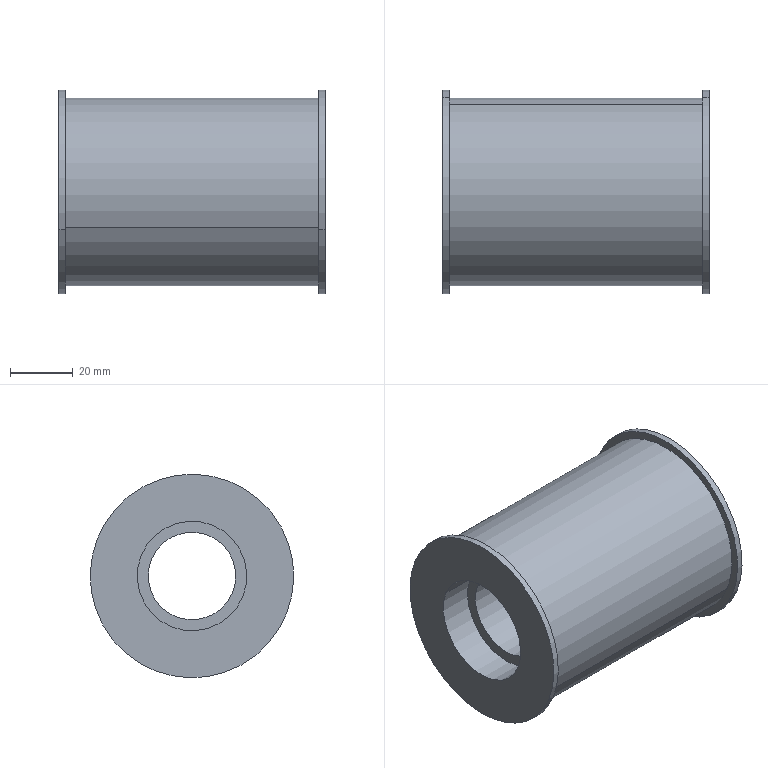Component | SolidWorks | ElectricalBoxAssembly2-1_AuxiliaryWheel-1 | 1 solid | 18 faces | box 85 x 65 x 65 mm | volume 182336 mm3 | cylinder 12 | plane 6 | commonest cylinder face diameters 35 x4 65 x4 28 x2 60 x2
build123d program:
from build123d import *


with BuildPart() as part:
    # Sketch1 → Revolve1 (revolve)
    with BuildSketch(Plane(origin=(0, 0, 0), x_dir=(1, 0, 0), z_dir=(0, 1, 0)), mode=Mode.PRIVATE) as revolve1_sk:
        Polygon((0, 17.5), (0, 32.5), (2, 32.5), (2, 30), (83, 30), (83, 32.5), (85, 32.5), (85, 17.5), (74, 17.5), (74, 14), (11, 14), (11, 17.5), align=None)
    revolve(revolve1_sk.sketch.rotate(Axis((-16.25, 0, 0), (1, 0, 0)), 180), axis=Axis((-16.25, 0, 0), (1, 0, 0)))


solid = part.part

# Placed as in the assembly
solid = solid.moved(Location((645.968, 334.666, 1526.399), (0, 0, 0)))
STEP:
#1=COLOUR_RGB('',0.7922,0.8196,0.9333);
#2=FILL_AREA_STYLE_COLOUR('',#1);
#3=FILL_AREA_STYLE('',(#2));
#4=SURFACE_STYLE_FILL_AREA(#3);
#5=SURFACE_SIDE_STYLE('',(#4));
#6=SURFACE_STYLE_USAGE(.BOTH.,#5);
#7=PRESENTATION_STYLE_ASSIGNMENT((#6));
#8=CARTESIAN_POINT('',(25.865,13.815,60.351));
#9=VERTEX_POINT('',#8);
#10=CARTESIAN_POINT('',(25.865,12.537,59.838));
#11=VERTEX_POINT('',#10);
#12=CARTESIAN_POINT('',(25.865,13.176,60.094));
#13=DIRECTION('',(-1.,-0.,-0.));
#14=DIRECTION('',(0.,-0.9279,-0.3728));
#15=AXIS2_PLACEMENT_3D('',#12,#13,#14);
#16=CIRCLE('',#15,0.689);
#17=EDGE_CURVE('',#9,#11,#16,.T.);
#18=ORIENTED_EDGE('',*,*,#17,.F.);
#19=CARTESIAN_POINT('',(25.432,13.815,60.351));
#20=VERTEX_POINT('',#19);
#21=CARTESIAN_POINT('',(24.792,13.815,60.351));
#22=DIRECTION('',(-1.,-0.,-0.));
#23=VECTOR('',#22,39.37);
#24=LINE('',#21,#23);
#25=EDGE_CURVE('',#9,#20,#24,.T.);
#26=ORIENTED_EDGE('',*,*,#25,.T.);
#27=CARTESIAN_POINT('',(25.432,12.537,59.838));
#28=VERTEX_POINT('',#27);
#29=CARTESIAN_POINT('',(25.432,13.176,60.094));
#30=DIRECTION('',(-1.,-0.,-0.));
#31=DIRECTION('',(0.,-0.9279,-0.3728));
#32=AXIS2_PLACEMENT_3D('',#29,#30,#31);
#33=CIRCLE('',#32,0.689);
#34=EDGE_CURVE('',#20,#28,#33,.T.);
#35=ORIENTED_EDGE('',*,*,#34,.T.);
#36=CARTESIAN_POINT('',(24.792,12.537,59.838));
#37=DIRECTION('',(-1.,-0.,-0.));
#38=VECTOR('',#37,39.37);
#39=LINE('',#36,#38);
#40=EDGE_CURVE('',#11,#28,#39,.T.);
#41=ORIENTED_EDGE('',*,*,#40,.F.);
#42=EDGE_LOOP('',(#18,#26,#35,#41));
#43=FACE_OUTER_BOUND('',#42,.T.);
#44=CARTESIAN_POINT('',(24.792,13.176,60.094));
#45=DIRECTION('',(-1.,-0.,-0.));
#46=DIRECTION('',(0.,-0.9279,-0.3728));
#47=AXIS2_PLACEMENT_3D('',#44,#45,#46);
#48=CYLINDRICAL_SURFACE('',#47,0.689);
#49=ADVANCED_FACE('',(#43),#48,.F.);
#50=CARTESIAN_POINT('',(28.345,13.687,60.3));
#51=VERTEX_POINT('',#50);
#52=CARTESIAN_POINT('',(28.345,12.664,59.889));
#53=VERTEX_POINT('',#52);
#54=CARTESIAN_POINT('',(28.345,13.176,60.094));
#55=DIRECTION('',(-1.,-0.,-0.));
#56=DIRECTION('',(0.,-0.9279,-0.3728));
#57=AXIS2_PLACEMENT_3D('',#54,#55,#56);
#58=CIRCLE('',#57,0.5512);
#59=EDGE_CURVE('',#51,#53,#58,.T.);
#60=ORIENTED_EDGE('',*,*,#59,.F.);
#61=CARTESIAN_POINT('',(25.865,13.687,60.3));
#62=VERTEX_POINT('',#61);
#63=CARTESIAN_POINT('',(24.792,13.687,60.3));
#64=DIRECTION('',(-1.,-0.,-0.));
#65=VECTOR('',#64,39.37);
#66=LINE('',#63,#65);
#67=EDGE_CURVE('',#51,#62,#66,.T.);
#68=ORIENTED_EDGE('',*,*,#67,.T.);
#69=CARTESIAN_POINT('',(25.865,12.664,59.889));
#70=VERTEX_POINT('',#69);
#71=CARTESIAN_POINT('',(25.865,13.176,60.094));
#72=DIRECTION('',(-1.,-0.,-0.));
#73=DIRECTION('',(0.,-0.9279,-0.3728));
#74=AXIS2_PLACEMENT_3D('',#71,#72,#73);
#75=CIRCLE('',#74,0.5512);
#76=EDGE_CURVE('',#62,#70,#75,.T.);
#77=ORIENTED_EDGE('',*,*,#76,.T.);
#78=CARTESIAN_POINT('',(24.792,12.664,59.889));
#79=DIRECTION('',(-1.,-0.,-0.));
#80=VECTOR('',#79,39.37);
#81=LINE('',#78,#80);
#82=EDGE_CURVE('',#53,#70,#81,.T.);
#83=ORIENTED_EDGE('',*,*,#82,.F.);
#84=EDGE_LOOP('',(#60,#68,#77,#83));
#85=FACE_OUTER_BOUND('',#84,.T.);
#86=CARTESIAN_POINT('',(24.792,13.176,60.094));
#87=DIRECTION('',(-1.,-0.,-0.));
#88=DIRECTION('',(0.,-0.9279,-0.3728));
#89=AXIS2_PLACEMENT_3D('',#86,#87,#88);
#90=CYLINDRICAL_SURFACE('',#89,0.5512);
#91=ADVANCED_FACE('',(#85),#90,.F.);
#92=CARTESIAN_POINT('',(28.778,13.815,60.351));
#93=VERTEX_POINT('',#92);
#94=CARTESIAN_POINT('',(28.778,12.537,59.838));
#95=VERTEX_POINT('',#94);
#96=CARTESIAN_POINT('',(28.778,13.176,60.094));
#97=DIRECTION('',(-1.,-0.,-0.));
#98=DIRECTION('',(0.,-0.9279,-0.3728));
#99=AXIS2_PLACEMENT_3D('',#96,#97,#98);
#100=CIRCLE('',#99,0.689);
#101=EDGE_CURVE('',#93,#95,#100,.T.);
#102=ORIENTED_EDGE('',*,*,#101,.F.);
#103=CARTESIAN_POINT('',(28.345,13.815,60.351));
#104=VERTEX_POINT('',#103);
#105=CARTESIAN_POINT('',(24.792,13.815,60.351));
#106=DIRECTION('',(-1.,-0.,-0.));
#107=VECTOR('',#106,39.37);
#108=LINE('',#105,#107);
#109=EDGE_CURVE('',#93,#104,#108,.T.);
#110=ORIENTED_EDGE('',*,*,#109,.T.);
#111=CARTESIAN_POINT('',(28.345,12.537,59.838));
#112=VERTEX_POINT('',#111);
#113=CARTESIAN_POINT('',(28.345,13.176,60.094));
#114=DIRECTION('',(-1.,-0.,-0.));
#115=DIRECTION('',(0.,-0.9279,-0.3728));
#116=AXIS2_PLACEMENT_3D('',#113,#114,#115);
#117=CIRCLE('',#116,0.689);
#118=EDGE_CURVE('',#104,#112,#117,.T.);
#119=ORIENTED_EDGE('',*,*,#118,.T.);
#120=CARTESIAN_POINT('',(24.792,12.537,59.838));
#121=DIRECTION('',(-1.,-0.,-0.));
#122=VECTOR('',#121,39.37);
#123=LINE('',#120,#122);
#124=EDGE_CURVE('',#95,#112,#123,.T.);
#125=ORIENTED_EDGE('',*,*,#124,.F.);
#126=EDGE_LOOP('',(#102,#110,#119,#125));
#127=FACE_OUTER_BOUND('',#126,.T.);
#128=CARTESIAN_POINT('',(24.792,13.176,60.094));
#129=DIRECTION('',(-1.,-0.,-0.));
#130=DIRECTION('',(0.,-0.9279,-0.3728));
#131=AXIS2_PLACEMENT_3D('',#128,#129,#130);
#132=CYLINDRICAL_SURFACE('',#131,0.689);
#133=ADVANCED_FACE('',(#127),#132,.F.);
#134=CARTESIAN_POINT('',(28.778,11.989,59.617));
#135=VERTEX_POINT('',#134);
#136=CARTESIAN_POINT('',(28.778,14.363,60.571));
#137=VERTEX_POINT('',#136);
#138=CARTESIAN_POINT('',(28.778,13.176,60.094));
#139=DIRECTION('',(-1.,-0.,-0.));
#140=DIRECTION('',(0.,-0.9279,-0.3728));
#141=AXIS2_PLACEMENT_3D('',#138,#139,#140);
#142=CIRCLE('',#141,1.28);
#143=EDGE_CURVE('',#135,#137,#142,.T.);
#144=ORIENTED_EDGE('',*,*,#143,.T.);
#145=CARTESIAN_POINT('',(28.7,14.363,60.571));
#146=VERTEX_POINT('',#145);
#147=CARTESIAN_POINT('',(24.792,14.363,60.571));
#148=DIRECTION('',(-1.,-0.,-0.));
#149=VECTOR('',#148,39.37);
#150=LINE('',#147,#149);
#151=EDGE_CURVE('',#137,#146,#150,.T.);
#152=ORIENTED_EDGE('',*,*,#151,.T.);
#153=CARTESIAN_POINT('',(28.7,11.989,59.617));
#154=VERTEX_POINT('',#153);
#155=CARTESIAN_POINT('',(28.7,13.176,60.094));
#156=DIRECTION('',(-1.,-0.,-0.));
#157=DIRECTION('',(0.,-0.9279,-0.3728));
#158=AXIS2_PLACEMENT_3D('',#155,#156,#157);
#159=CIRCLE('',#158,1.28);
#160=EDGE_CURVE('',#154,#146,#159,.T.);
#161=ORIENTED_EDGE('',*,*,#160,.F.);
#162=CARTESIAN_POINT('',(24.792,11.989,59.617));
#163=DIRECTION('',(-1.,-0.,-0.));
#164=VECTOR('',#163,39.37);
#165=LINE('',#162,#164);
#166=EDGE_CURVE('',#135,#154,#165,.T.);
#167=ORIENTED_EDGE('',*,*,#166,.F.);
#168=EDGE_LOOP('',(#144,#152,#161,#167));
#169=FACE_OUTER_BOUND('',#168,.T.);
#170=CARTESIAN_POINT('',(24.792,13.176,60.094));
#171=DIRECTION('',(-1.,-0.,-0.));
#172=DIRECTION('',(0.,-0.9279,-0.3728));
#173=AXIS2_PLACEMENT_3D('',#170,#171,#172);
#174=CYLINDRICAL_SURFACE('',#173,1.28);
#175=ADVANCED_FACE('',(#169),#174,.T.);
#176=CARTESIAN_POINT('',(28.7,12.08,59.654));
#177=VERTEX_POINT('',#176);
#178=CARTESIAN_POINT('',(28.7,14.272,60.535));
#179=VERTEX_POINT('',#178);
#180=CARTESIAN_POINT('',(28.7,13.176,60.094));
#181=DIRECTION('',(-1.,-0.,-0.));
#182=DIRECTION('',(0.,-0.9279,-0.3728));
#183=AXIS2_PLACEMENT_3D('',#180,#181,#182);
#184=CIRCLE('',#183,1.181);
#185=EDGE_CURVE('',#177,#179,#184,.T.);
#186=ORIENTED_EDGE('',*,*,#185,.T.);
#187=CARTESIAN_POINT('',(25.511,14.272,60.535));
#188=VERTEX_POINT('',#187);
#189=CARTESIAN_POINT('',(24.792,14.272,60.535));
#190=DIRECTION('',(-1.,-0.,-0.));
#191=VECTOR('',#190,39.37);
#192=LINE('',#189,#191);
#193=EDGE_CURVE('',#179,#188,#192,.T.);
#194=ORIENTED_EDGE('',*,*,#193,.T.);
#195=CARTESIAN_POINT('',(25.511,12.08,59.654));
#196=VERTEX_POINT('',#195);
#197=CARTESIAN_POINT('',(25.511,13.176,60.094));
#198=DIRECTION('',(-1.,-0.,-0.));
#199=DIRECTION('',(0.,-0.9279,-0.3728));
#200=AXIS2_PLACEMENT_3D('',#197,#198,#199);
#201=CIRCLE('',#200,1.181);
#202=EDGE_CURVE('',#196,#188,#201,.T.);
#203=ORIENTED_EDGE('',*,*,#202,.F.);
#204=CARTESIAN_POINT('',(24.792,12.08,59.654));
#205=DIRECTION('',(-1.,-0.,-0.));
#206=VECTOR('',#205,39.37);
#207=LINE('',#204,#206);
#208=EDGE_CURVE('',#177,#196,#207,.T.);
#209=ORIENTED_EDGE('',*,*,#208,.F.);
#210=EDGE_LOOP('',(#186,#194,#203,#209));
#211=FACE_OUTER_BOUND('',#210,.T.);
#212=CARTESIAN_POINT('',(24.792,13.176,60.094));
#213=DIRECTION('',(-1.,-0.,-0.));
#214=DIRECTION('',(0.,-0.9279,-0.3728));
#215=AXIS2_PLACEMENT_3D('',#212,#213,#214);
#216=CYLINDRICAL_SURFACE('',#215,1.181);
#217=ADVANCED_FACE('',(#211),#216,.T.);
#218=CARTESIAN_POINT('',(25.511,11.989,59.617));
#219=VERTEX_POINT('',#218);
#220=CARTESIAN_POINT('',(25.511,14.363,60.571));
#221=VERTEX_POINT('',#220);
#222=CARTESIAN_POINT('',(25.511,13.176,60.094));
#223=DIRECTION('',(-1.,-0.,-0.));
#224=DIRECTION('',(0.,-0.9279,-0.3728));
#225=AXIS2_PLACEMENT_3D('',#222,#223,#224);
#226=CIRCLE('',#225,1.28);
#227=EDGE_CURVE('',#219,#221,#226,.T.);
#228=ORIENTED_EDGE('',*,*,#227,.T.);
#229=CARTESIAN_POINT('',(25.432,14.363,60.571));
#230=VERTEX_POINT('',#229);
#231=CARTESIAN_POINT('',(24.792,14.363,60.571));
#232=DIRECTION('',(-1.,-0.,-0.));
#233=VECTOR('',#232,39.37);
#234=LINE('',#231,#233);
#235=EDGE_CURVE('',#221,#230,#234,.T.);
#236=ORIENTED_EDGE('',*,*,#235,.T.);
#237=CARTESIAN_POINT('',(25.432,11.989,59.617));
#238=VERTEX_POINT('',#237);
#239=CARTESIAN_POINT('',(25.432,13.176,60.094));
#240=DIRECTION('',(-1.,-0.,-0.));
#241=DIRECTION('',(0.,-0.9279,-0.3728));
#242=AXIS2_PLACEMENT_3D('',#239,#240,#241);
#243=CIRCLE('',#242,1.28);
#244=EDGE_CURVE('',#238,#230,#243,.T.);
#245=ORIENTED_EDGE('',*,*,#244,.F.);
#246=CARTESIAN_POINT('',(24.792,11.989,59.617));
#247=DIRECTION('',(-1.,-0.,-0.));
#248=VECTOR('',#247,39.37);
#249=LINE('',#246,#248);
#250=EDGE_CURVE('',#219,#238,#249,.T.);
#251=ORIENTED_EDGE('',*,*,#250,.F.);
#252=EDGE_LOOP('',(#228,#236,#245,#251));
#253=FACE_OUTER_BOUND('',#252,.T.);
#254=CARTESIAN_POINT('',(24.792,13.176,60.094));
#255=DIRECTION('',(-1.,-0.,-0.));
#256=DIRECTION('',(0.,-0.9279,-0.3728));
#257=AXIS2_PLACEMENT_3D('',#254,#255,#256);
#258=CYLINDRICAL_SURFACE('',#257,1.28);
#259=ADVANCED_FACE('',(#253),#258,.T.);
#260=ORIENTED_EDGE('',*,*,#235,.F.);
#261=CARTESIAN_POINT('',(25.511,13.176,60.094));
#262=DIRECTION('',(-1.,-0.,-0.));
#263=DIRECTION('',(0.,-0.9279,-0.3728));
#264=AXIS2_PLACEMENT_3D('',#261,#262,#263);
#265=CIRCLE('',#264,1.28);
#266=EDGE_CURVE('',#221,#219,#265,.T.);
#267=ORIENTED_EDGE('',*,*,#266,.T.);
#268=ORIENTED_EDGE('',*,*,#250,.T.);
#269=CARTESIAN_POINT('',(25.432,13.176,60.094));
#270=DIRECTION('',(-1.,-0.,-0.));
#271=DIRECTION('',(0.,-0.9279,-0.3728));
#272=AXIS2_PLACEMENT_3D('',#269,#270,#271);
#273=CIRCLE('',#272,1.28);
#274=EDGE_CURVE('',#230,#238,#273,.T.);
#275=ORIENTED_EDGE('',*,*,#274,.F.);
#276=EDGE_LOOP('',(#260,#267,#268,#275));
#277=FACE_OUTER_BOUND('',#276,.T.);
#278=CARTESIAN_POINT('',(24.792,13.176,60.094));
#279=DIRECTION('',(-1.,-0.,-0.));
#280=DIRECTION('',(0.,-0.9279,-0.3728));
#281=AXIS2_PLACEMENT_3D('',#278,#279,#280);
#282=CYLINDRICAL_SURFACE('',#281,1.28);
#283=ADVANCED_FACE('',(#277),#282,.T.);
#284=ORIENTED_EDGE('',*,*,#227,.F.);
#285=ORIENTED_EDGE('',*,*,#266,.F.);
#286=EDGE_LOOP('',(#284,#285));
#287=FACE_OUTER_BOUND('',#286,.T.);
#288=ORIENTED_EDGE('',*,*,#202,.T.);
#289=CARTESIAN_POINT('',(25.511,13.176,60.094));
#290=DIRECTION('',(-1.,-0.,-0.));
#291=DIRECTION('',(0.,-0.9279,-0.3728));
#292=AXIS2_PLACEMENT_3D('',#289,#290,#291);
#293=CIRCLE('',#292,1.181);
#294=EDGE_CURVE('',#188,#196,#293,.T.);
#295=ORIENTED_EDGE('',*,*,#294,.T.);
#296=EDGE_LOOP('',(#288,#295));
#297=FACE_BOUND('',#296,.T.);
#298=CARTESIAN_POINT('',(25.511,14.363,60.571));
#299=DIRECTION('',(-1.,-0.,-0.));
#300=DIRECTION('',(0.,-0.9279,-0.3728));
#301=AXIS2_PLACEMENT_3D('',#298,#299,#300);
#302=PLANE('',#301);
#303=ADVANCED_FACE('',(#287,#297),#302,.F.);
#304=ORIENTED_EDGE('',*,*,#193,.F.);
#305=CARTESIAN_POINT('',(28.7,13.176,60.094));
#306=DIRECTION('',(-1.,-0.,-0.));
#307=DIRECTION('',(0.,-0.9279,-0.3728));
#308=AXIS2_PLACEMENT_3D('',#305,#306,#307);
#309=CIRCLE('',#308,1.181);
#310=EDGE_CURVE('',#179,#177,#309,.T.);
#311=ORIENTED_EDGE('',*,*,#310,.T.);
#312=ORIENTED_EDGE('',*,*,#208,.T.);
#313=ORIENTED_EDGE('',*,*,#294,.F.);
#314=EDGE_LOOP('',(#304,#311,#312,#313));
#315=FACE_OUTER_BOUND('',#314,.T.);
#316=CARTESIAN_POINT('',(24.792,13.176,60.094));
#317=DIRECTION('',(-1.,-0.,-0.));
#318=DIRECTION('',(0.,-0.9279,-0.3728));
#319=AXIS2_PLACEMENT_3D('',#316,#317,#318);
#320=CYLINDRICAL_SURFACE('',#319,1.181);
#321=ADVANCED_FACE('',(#315),#320,.T.);
#322=ORIENTED_EDGE('',*,*,#185,.F.);
#323=ORIENTED_EDGE('',*,*,#310,.F.);
#324=EDGE_LOOP('',(#322,#323));
#325=FACE_BOUND('',#324,.T.);
#326=ORIENTED_EDGE('',*,*,#160,.T.);
#327=CARTESIAN_POINT('',(28.7,13.176,60.094));
#328=DIRECTION('',(-1.,-0.,-0.));
#329=DIRECTION('',(0.,-0.9279,-0.3728));
#330=AXIS2_PLACEMENT_3D('',#327,#328,#329);
#331=CIRCLE('',#330,1.28);
#332=EDGE_CURVE('',#146,#154,#331,.T.);
#333=ORIENTED_EDGE('',*,*,#332,.T.);
#334=EDGE_LOOP('',(#326,#333));
#335=FACE_OUTER_BOUND('',#334,.T.);
#336=CARTESIAN_POINT('',(28.7,14.272,60.535));
#337=DIRECTION('',(1.,0.,0.));
#338=DIRECTION('',(-0.,0.9279,0.3728));
#339=AXIS2_PLACEMENT_3D('',#336,#337,#338);
#340=PLANE('',#339);
#341=ADVANCED_FACE('',(#325,#335),#340,.F.);
#342=ORIENTED_EDGE('',*,*,#151,.F.);
#343=CARTESIAN_POINT('',(28.778,13.176,60.094));
#344=DIRECTION('',(-1.,-0.,-0.));
#345=DIRECTION('',(0.,-0.9279,-0.3728));
#346=AXIS2_PLACEMENT_3D('',#343,#344,#345);
#347=CIRCLE('',#346,1.28);
#348=EDGE_CURVE('',#137,#135,#347,.T.);
#349=ORIENTED_EDGE('',*,*,#348,.T.);
#350=ORIENTED_EDGE('',*,*,#166,.T.);
#351=ORIENTED_EDGE('',*,*,#332,.F.);
#352=EDGE_LOOP('',(#342,#349,#350,#351));
#353=FACE_OUTER_BOUND('',#352,.T.);
#354=CARTESIAN_POINT('',(24.792,13.176,60.094));
#355=DIRECTION('',(-1.,-0.,-0.));
#356=DIRECTION('',(0.,-0.9279,-0.3728));
#357=AXIS2_PLACEMENT_3D('',#354,#355,#356);
#358=CYLINDRICAL_SURFACE('',#357,1.28);
#359=ADVANCED_FACE('',(#353),#358,.T.);
#360=ORIENTED_EDGE('',*,*,#143,.F.);
#361=ORIENTED_EDGE('',*,*,#348,.F.);
#362=EDGE_LOOP('',(#360,#361));
#363=FACE_OUTER_BOUND('',#362,.T.);
#364=CARTESIAN_POINT('',(28.778,13.176,60.094));
#365=DIRECTION('',(-1.,-0.,-0.));
#366=DIRECTION('',(0.,-0.9279,-0.3728));
#367=AXIS2_PLACEMENT_3D('',#364,#365,#366);
#368=CIRCLE('',#367,0.689);
#369=EDGE_CURVE('',#95,#93,#368,.T.);
#370=ORIENTED_EDGE('',*,*,#369,.T.);
#371=ORIENTED_EDGE('',*,*,#101,.T.);
#372=EDGE_LOOP('',(#370,#371));
#373=FACE_BOUND('',#372,.T.);
#374=CARTESIAN_POINT('',(28.778,14.363,60.571));
#375=DIRECTION('',(-1.,-0.,-0.));
#376=DIRECTION('',(0.,-0.9279,-0.3728));
#377=AXIS2_PLACEMENT_3D('',#374,#375,#376);
#378=PLANE('',#377);
#379=ADVANCED_FACE('',(#363,#373),#378,.F.);
#380=ORIENTED_EDGE('',*,*,#109,.F.);
#381=ORIENTED_EDGE('',*,*,#369,.F.);
#382=ORIENTED_EDGE('',*,*,#124,.T.);
#383=CARTESIAN_POINT('',(28.345,13.176,60.094));
#384=DIRECTION('',(-1.,-0.,-0.));
#385=DIRECTION('',(0.,-0.9279,-0.3728));
#386=AXIS2_PLACEMENT_3D('',#383,#384,#385);
#387=CIRCLE('',#386,0.689);
#388=EDGE_CURVE('',#112,#104,#387,.T.);
#389=ORIENTED_EDGE('',*,*,#388,.T.);
#390=EDGE_LOOP('',(#380,#381,#382,#389));
#391=FACE_OUTER_BOUND('',#390,.T.);
#392=CARTESIAN_POINT('',(24.792,13.176,60.094));
#393=DIRECTION('',(-1.,-0.,-0.));
#394=DIRECTION('',(0.,-0.9279,-0.3728));
#395=AXIS2_PLACEMENT_3D('',#392,#393,#394);
#396=CYLINDRICAL_SURFACE('',#395,0.689);
#397=ADVANCED_FACE('',(#391),#396,.F.);
#398=ORIENTED_EDGE('',*,*,#388,.F.);
#399=ORIENTED_EDGE('',*,*,#118,.F.);
#400=EDGE_LOOP('',(#398,#399));
#401=FACE_OUTER_BOUND('',#400,.T.);
#402=CARTESIAN_POINT('',(28.345,13.176,60.094));
#403=DIRECTION('',(-1.,-0.,-0.));
#404=DIRECTION('',(0.,-0.9279,-0.3728));
#405=AXIS2_PLACEMENT_3D('',#402,#403,#404);
#406=CIRCLE('',#405,0.5512);
#407=EDGE_CURVE('',#53,#51,#406,.T.);
#408=ORIENTED_EDGE('',*,*,#407,.T.);
#409=ORIENTED_EDGE('',*,*,#59,.T.);
#410=EDGE_LOOP('',(#408,#409));
#411=FACE_BOUND('',#410,.T.);
#412=CARTESIAN_POINT('',(28.345,13.815,60.351));
#413=DIRECTION('',(-1.,-0.,-0.));
#414=DIRECTION('',(0.,-0.9279,-0.3728));
#415=AXIS2_PLACEMENT_3D('',#412,#413,#414);
#416=PLANE('',#415);
#417=ADVANCED_FACE('',(#401,#411),#416,.F.);
#418=ORIENTED_EDGE('',*,*,#67,.F.);
#419=ORIENTED_EDGE('',*,*,#407,.F.);
#420=ORIENTED_EDGE('',*,*,#82,.T.);
#421=CARTESIAN_POINT('',(25.865,13.176,60.094));
#422=DIRECTION('',(-1.,-0.,-0.));
#423=DIRECTION('',(0.,-0.9279,-0.3728));
#424=AXIS2_PLACEMENT_3D('',#421,#422,#423);
#425=CIRCLE('',#424,0.5512);
#426=EDGE_CURVE('',#70,#62,#425,.T.);
#427=ORIENTED_EDGE('',*,*,#426,.T.);
#428=EDGE_LOOP('',(#418,#419,#420,#427));
#429=FACE_OUTER_BOUND('',#428,.T.);
#430=CARTESIAN_POINT('',(24.792,13.176,60.094));
#431=DIRECTION('',(-1.,-0.,-0.));
#432=DIRECTION('',(0.,-0.9279,-0.3728));
#433=AXIS2_PLACEMENT_3D('',#430,#431,#432);
#434=CYLINDRICAL_SURFACE('',#433,0.5512);
#435=ADVANCED_FACE('',(#429),#434,.F.);
#436=ORIENTED_EDGE('',*,*,#426,.F.);
#437=ORIENTED_EDGE('',*,*,#76,.F.);
#438=EDGE_LOOP('',(#436,#437));
#439=FACE_BOUND('',#438,.T.);
#440=CARTESIAN_POINT('',(25.865,13.176,60.094));
#441=DIRECTION('',(-1.,-0.,-0.));
#442=DIRECTION('',(0.,-0.9279,-0.3728));
#443=AXIS2_PLACEMENT_3D('',#440,#441,#442);
#444=CIRCLE('',#443,0.689);
#445=EDGE_CURVE('',#11,#9,#444,.T.);
#446=ORIENTED_EDGE('',*,*,#445,.T.);
#447=ORIENTED_EDGE('',*,*,#17,.T.);
#448=EDGE_LOOP('',(#446,#447));
#449=FACE_OUTER_BOUND('',#448,.T.);
#450=CARTESIAN_POINT('',(25.865,13.815,60.351));
#451=DIRECTION('',(1.,0.,0.));
#452=DIRECTION('',(-0.,0.9279,0.3728));
#453=AXIS2_PLACEMENT_3D('',#450,#451,#452);
#454=PLANE('',#453);
#455=ADVANCED_FACE('',(#439,#449),#454,.F.);
#456=ORIENTED_EDGE('',*,*,#25,.F.);
#457=ORIENTED_EDGE('',*,*,#445,.F.);
#458=ORIENTED_EDGE('',*,*,#40,.T.);
#459=CARTESIAN_POINT('',(25.432,13.176,60.094));
#460=DIRECTION('',(-1.,-0.,-0.));
#461=DIRECTION('',(0.,-0.9279,-0.3728));
#462=AXIS2_PLACEMENT_3D('',#459,#460,#461);
#463=CIRCLE('',#462,0.689);
#464=EDGE_CURVE('',#28,#20,#463,.T.);
#465=ORIENTED_EDGE('',*,*,#464,.T.);
#466=EDGE_LOOP('',(#456,#457,#458,#465));
#467=FACE_OUTER_BOUND('',#466,.T.);
#468=CARTESIAN_POINT('',(24.792,13.176,60.094));
#469=DIRECTION('',(-1.,-0.,-0.));
#470=DIRECTION('',(0.,-0.9279,-0.3728));
#471=AXIS2_PLACEMENT_3D('',#468,#469,#470);
#472=CYLINDRICAL_SURFACE('',#471,0.689);
#473=ADVANCED_FACE('',(#467),#472,.F.);
#474=ORIENTED_EDGE('',*,*,#464,.F.);
#475=ORIENTED_EDGE('',*,*,#34,.F.);
#476=EDGE_LOOP('',(#474,#475));
#477=FACE_BOUND('',#476,.T.);
#478=ORIENTED_EDGE('',*,*,#244,.T.);
#479=ORIENTED_EDGE('',*,*,#274,.T.);
#480=EDGE_LOOP('',(#478,#479));
#481=FACE_OUTER_BOUND('',#480,.T.);
#482=CARTESIAN_POINT('',(25.432,13.815,60.351));
#483=DIRECTION('',(1.,0.,0.));
#484=DIRECTION('',(-0.,0.9279,0.3728));
#485=AXIS2_PLACEMENT_3D('',#482,#483,#484);
#486=PLANE('',#485);
#487=ADVANCED_FACE('',(#477,#481),#486,.F.);
#488=CLOSED_SHELL('',(#49,#91,#133,#175,#217,#259,#283,#303,#321,#341,#359,#379,#397,#417,#435,#455,#473,#487));
#489=MANIFOLD_SOLID_BREP('',#488);
#490=STYLED_ITEM('',(#7),#489);
#491=PRESENTATION_LAYER_ASSIGNMENT('','',(#490));
#492=CARTESIAN_POINT('',(0.,0.,0.));
#493=DIRECTION('',(0.,0.,1.));
#494=DIRECTION('',(1.,0.,0.));
#495=AXIS2_PLACEMENT_3D('',#492,#493,#494);
#496=(LENGTH_UNIT()NAMED_UNIT(*)SI_UNIT($,.METRE.));
#497=LENGTH_MEASURE_WITH_UNIT(LENGTH_MEASURE(0.0254),#496);
#498=DIMENSIONAL_EXPONENTS(1.,0.,0.,0.,0.,0.,0.);
#499=(CONVERSION_BASED_UNIT('',#497)LENGTH_UNIT()NAMED_UNIT(#498));
#500=UNCERTAINTY_MEASURE_WITH_UNIT(LENGTH_MEASURE(0.00001),#499,'','');
#501=(NAMED_UNIT(*)PLANE_ANGLE_UNIT()SI_UNIT($,.RADIAN.));
#502=(NAMED_UNIT(*)SI_UNIT($,.STERADIAN.)SOLID_ANGLE_UNIT());
#503=(GEOMETRIC_REPRESENTATION_CONTEXT(3)GLOBAL_UNCERTAINTY_ASSIGNED_CONTEXT((#500))GLOBAL_UNIT_ASSIGNED_CONTEXT((#499,#501,#502))REPRESENTATION_CONTEXT('',''));
#504=ADVANCED_BREP_SHAPE_REPRESENTATION('',(#489,#495),#503);
#505=(LENGTH_UNIT()NAMED_UNIT(*)SI_UNIT($,.METRE.));
#506=LENGTH_MEASURE_WITH_UNIT(LENGTH_MEASURE(0.0254),#505);
#507=DIMENSIONAL_EXPONENTS(1.,0.,0.,0.,0.,0.,0.);
#508=(CONVERSION_BASED_UNIT('',#506)LENGTH_UNIT()NAMED_UNIT(#507));
#509=UNCERTAINTY_MEASURE_WITH_UNIT(LENGTH_MEASURE(0.00001),#508,'','');
#510=(NAMED_UNIT(*)PLANE_ANGLE_UNIT()SI_UNIT($,.RADIAN.));
#511=(NAMED_UNIT(*)SI_UNIT($,.STERADIAN.)SOLID_ANGLE_UNIT());
#512=(GEOMETRIC_REPRESENTATION_CONTEXT(3)GLOBAL_UNCERTAINTY_ASSIGNED_CONTEXT((#509))GLOBAL_UNIT_ASSIGNED_CONTEXT((#508,#510,#511))REPRESENTATION_CONTEXT('',''));
#513=MECHANICAL_DESIGN_GEOMETRIC_PRESENTATION_REPRESENTATION('',(#490),#512);